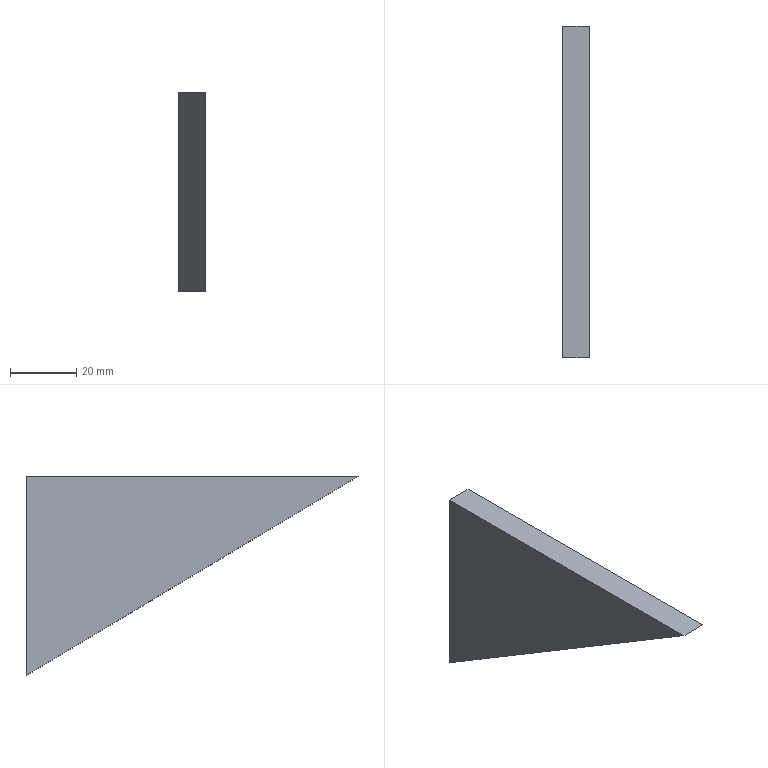Component | SolidWorks | NewTypeCurveBenderReducerPlate-DoubleWheel-2_NewCurveBender(New)Triangle-DoubleWheel-1 | 1 solid | 5 faces | box 8 x 100 x 60 mm | volume 24000 mm3 | plane 5
build123d program:
from build123d import *

# Parameters (mm, degrees)
BOSS_EXTRUDE1_DEPTH = 8


with BuildPart() as part:
    # Sketch1 → Boss-Extrude1 (new body)
    with BuildSketch(Plane.XY):
        Polygon((0, 0), (-60, 0), (0, 100), align=None)
    extrude(amount=BOSS_EXTRUDE1_DEPTH)


solid = part.part

# Placed as in the assembly
solid = solid.moved(Location((77, 8, 192), (180, 90, 0)))
STEP:
#1=COLOUR_RGB('',0.7922,0.8196,0.9333);
#2=FILL_AREA_STYLE_COLOUR('',#1);
#3=FILL_AREA_STYLE('',(#2));
#4=SURFACE_STYLE_FILL_AREA(#3);
#5=SURFACE_SIDE_STYLE('',(#4));
#6=SURFACE_STYLE_USAGE(.BOTH.,#5);
#7=PRESENTATION_STYLE_ASSIGNMENT((#6));
#8=CARTESIAN_POINT('',(3.031,0.315,7.559));
#9=VERTEX_POINT('',#8);
#10=CARTESIAN_POINT('',(3.031,-3.622,7.559));
#11=VERTEX_POINT('',#10);
#12=CARTESIAN_POINT('',(3.031,0.315,7.559));
#13=DIRECTION('',(-0.,-1.,-0.));
#14=VECTOR('',#13,39.37);
#15=LINE('',#12,#14);
#16=EDGE_CURVE('',#9,#11,#15,.T.);
#17=ORIENTED_EDGE('',*,*,#16,.T.);
#18=CARTESIAN_POINT('',(3.346,-3.622,7.559));
#19=VERTEX_POINT('',#18);
#20=CARTESIAN_POINT('',(3.346,-3.622,7.559));
#21=DIRECTION('',(-1.,0.,-0.));
#22=VECTOR('',#21,39.37);
#23=LINE('',#20,#22);
#24=EDGE_CURVE('',#19,#11,#23,.T.);
#25=ORIENTED_EDGE('',*,*,#24,.F.);
#26=CARTESIAN_POINT('',(3.346,0.315,7.559));
#27=VERTEX_POINT('',#26);
#28=CARTESIAN_POINT('',(3.346,0.315,7.559));
#29=DIRECTION('',(-0.,-1.,-0.));
#30=VECTOR('',#29,39.37);
#31=LINE('',#28,#30);
#32=EDGE_CURVE('',#27,#19,#31,.T.);
#33=ORIENTED_EDGE('',*,*,#32,.F.);
#34=CARTESIAN_POINT('',(3.346,0.315,7.559));
#35=DIRECTION('',(-1.,0.,-0.));
#36=VECTOR('',#35,39.37);
#37=LINE('',#34,#36);
#38=EDGE_CURVE('',#27,#9,#37,.T.);
#39=ORIENTED_EDGE('',*,*,#38,.T.);
#40=EDGE_LOOP('',(#17,#25,#33,#39));
#41=FACE_OUTER_BOUND('',#40,.T.);
#42=CARTESIAN_POINT('',(3.346,0.315,7.559));
#43=DIRECTION('',(0.,0.,-1.));
#44=DIRECTION('',(1.,-0.,0.));
#45=AXIS2_PLACEMENT_3D('',#42,#43,#44);
#46=PLANE('',#45);
#47=ADVANCED_FACE('',(#41),#46,.F.);
#48=CARTESIAN_POINT('',(3.031,0.315,5.197));
#49=VERTEX_POINT('',#48);
#50=CARTESIAN_POINT('',(3.031,-3.622,7.559));
#51=DIRECTION('',(0.,0.8575,-0.5145));
#52=VECTOR('',#51,39.37);
#53=LINE('',#50,#52);
#54=EDGE_CURVE('',#11,#49,#53,.T.);
#55=ORIENTED_EDGE('',*,*,#54,.T.);
#56=CARTESIAN_POINT('',(3.346,0.315,5.197));
#57=VERTEX_POINT('',#56);
#58=CARTESIAN_POINT('',(3.346,0.315,5.197));
#59=DIRECTION('',(-1.,0.,-0.));
#60=VECTOR('',#59,39.37);
#61=LINE('',#58,#60);
#62=EDGE_CURVE('',#57,#49,#61,.T.);
#63=ORIENTED_EDGE('',*,*,#62,.F.);
#64=CARTESIAN_POINT('',(3.346,-3.622,7.559));
#65=DIRECTION('',(0.,0.8575,-0.5145));
#66=VECTOR('',#65,39.37);
#67=LINE('',#64,#66);
#68=EDGE_CURVE('',#19,#57,#67,.T.);
#69=ORIENTED_EDGE('',*,*,#68,.F.);
#70=ORIENTED_EDGE('',*,*,#24,.T.);
#71=EDGE_LOOP('',(#55,#63,#69,#70));
#72=FACE_OUTER_BOUND('',#71,.T.);
#73=CARTESIAN_POINT('',(3.346,-3.622,7.559));
#74=DIRECTION('',(-0.,0.5145,0.8575));
#75=DIRECTION('',(-0.,-0.8575,0.5145));
#76=AXIS2_PLACEMENT_3D('',#73,#74,#75);
#77=PLANE('',#76);
#78=ADVANCED_FACE('',(#72),#77,.F.);
#79=CARTESIAN_POINT('',(3.031,0.315,7.559));
#80=DIRECTION('',(-0.,-0.,1.));
#81=VECTOR('',#80,39.37);
#82=LINE('',#79,#81);
#83=EDGE_CURVE('',#49,#9,#82,.T.);
#84=ORIENTED_EDGE('',*,*,#83,.T.);
#85=ORIENTED_EDGE('',*,*,#38,.F.);
#86=CARTESIAN_POINT('',(3.346,0.315,7.559));
#87=DIRECTION('',(-0.,-0.,1.));
#88=VECTOR('',#87,39.37);
#89=LINE('',#86,#88);
#90=EDGE_CURVE('',#57,#27,#89,.T.);
#91=ORIENTED_EDGE('',*,*,#90,.F.);
#92=ORIENTED_EDGE('',*,*,#62,.T.);
#93=EDGE_LOOP('',(#84,#85,#91,#92));
#94=FACE_OUTER_BOUND('',#93,.T.);
#95=CARTESIAN_POINT('',(3.346,0.315,7.559));
#96=DIRECTION('',(-0.,-1.,-0.));
#97=DIRECTION('',(1.,-0.,0.));
#98=AXIS2_PLACEMENT_3D('',#95,#96,#97);
#99=PLANE('',#98);
#100=ADVANCED_FACE('',(#94),#99,.F.);
#101=ORIENTED_EDGE('',*,*,#32,.T.);
#102=ORIENTED_EDGE('',*,*,#68,.T.);
#103=ORIENTED_EDGE('',*,*,#90,.T.);
#104=EDGE_LOOP('',(#101,#102,#103));
#105=FACE_OUTER_BOUND('',#104,.T.);
#106=CARTESIAN_POINT('',(3.346,0.315,7.559));
#107=DIRECTION('',(1.,-0.,0.));
#108=DIRECTION('',(-0.,-0.,1.));
#109=AXIS2_PLACEMENT_3D('',#106,#107,#108);
#110=PLANE('',#109);
#111=ADVANCED_FACE('',(#105),#110,.T.);
#112=ORIENTED_EDGE('',*,*,#16,.F.);
#113=ORIENTED_EDGE('',*,*,#83,.F.);
#114=ORIENTED_EDGE('',*,*,#54,.F.);
#115=EDGE_LOOP('',(#112,#113,#114));
#116=FACE_OUTER_BOUND('',#115,.T.);
#117=CARTESIAN_POINT('',(3.031,0.315,7.559));
#118=DIRECTION('',(1.,-0.,0.));
#119=DIRECTION('',(-0.,-0.,1.));
#120=AXIS2_PLACEMENT_3D('',#117,#118,#119);
#121=PLANE('',#120);
#122=ADVANCED_FACE('',(#116),#121,.F.);
#123=CLOSED_SHELL('',(#47,#78,#100,#111,#122));
#124=MANIFOLD_SOLID_BREP('',#123);
#125=STYLED_ITEM('',(#7),#124);
#126=(LENGTH_UNIT()NAMED_UNIT(*)SI_UNIT($,.METRE.));
#127=LENGTH_MEASURE_WITH_UNIT(LENGTH_MEASURE(0.0254),#126);
#128=DIMENSIONAL_EXPONENTS(1.,0.,0.,0.,0.,0.,0.);
#129=(CONVERSION_BASED_UNIT('',#127)LENGTH_UNIT()NAMED_UNIT(#128));
#130=UNCERTAINTY_MEASURE_WITH_UNIT(LENGTH_MEASURE(0.00001),#129,'','');
#131=(NAMED_UNIT(*)PLANE_ANGLE_UNIT()SI_UNIT($,.RADIAN.));
#132=(NAMED_UNIT(*)SI_UNIT($,.STERADIAN.)SOLID_ANGLE_UNIT());
#133=(GEOMETRIC_REPRESENTATION_CONTEXT(3)GLOBAL_UNCERTAINTY_ASSIGNED_CONTEXT((#130))GLOBAL_UNIT_ASSIGNED_CONTEXT((#129,#131,#132))REPRESENTATION_CONTEXT('',''));
#134=MECHANICAL_DESIGN_GEOMETRIC_PRESENTATION_REPRESENTATION('',(#125),#133);
#135=PRESENTATION_LAYER_ASSIGNMENT('','',(#125));
#136=CARTESIAN_POINT('',(0.,0.,0.));
#137=DIRECTION('',(0.,0.,1.));
#138=DIRECTION('',(1.,0.,0.));
#139=AXIS2_PLACEMENT_3D('',#136,#137,#138);
#140=(LENGTH_UNIT()NAMED_UNIT(*)SI_UNIT($,.METRE.));
#141=LENGTH_MEASURE_WITH_UNIT(LENGTH_MEASURE(0.0254),#140);
#142=DIMENSIONAL_EXPONENTS(1.,0.,0.,0.,0.,0.,0.);
#143=(CONVERSION_BASED_UNIT('',#141)LENGTH_UNIT()NAMED_UNIT(#142));
#144=UNCERTAINTY_MEASURE_WITH_UNIT(LENGTH_MEASURE(0.00001),#143,'','');
#145=(NAMED_UNIT(*)PLANE_ANGLE_UNIT()SI_UNIT($,.RADIAN.));
#146=(NAMED_UNIT(*)SI_UNIT($,.STERADIAN.)SOLID_ANGLE_UNIT());
#147=(GEOMETRIC_REPRESENTATION_CONTEXT(3)GLOBAL_UNCERTAINTY_ASSIGNED_CONTEXT((#144))GLOBAL_UNIT_ASSIGNED_CONTEXT((#143,#145,#146))REPRESENTATION_CONTEXT('',''));
#148=ADVANCED_BREP_SHAPE_REPRESENTATION('',(#124,#139),#147);